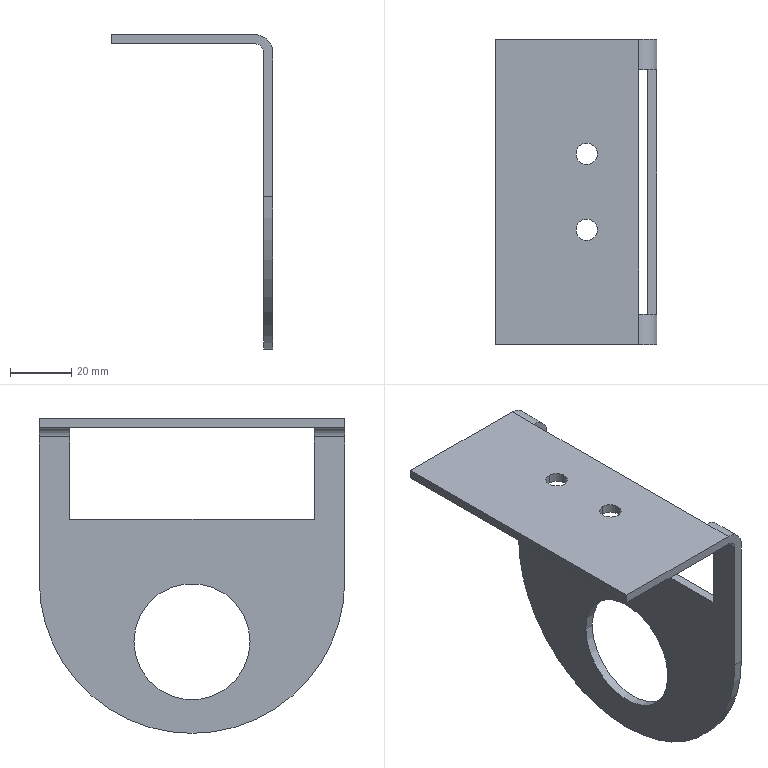Component | SolidWorks | PressureReducingValveHolder-1 | 1 solid | 23 faces | box 53 x 100 x 103 mm | volume 30292 mm3 | cylinder 12 | plane 11 | commonest cylinder face diameters 7 x4 38 x2 6 x2 12 x2 100 x2
STEP:
#1=COLOUR_RGB('',0.7922,0.8196,0.9333);
#2=FILL_AREA_STYLE_COLOUR('',#1);
#3=FILL_AREA_STYLE('',(#2));
#4=SURFACE_STYLE_FILL_AREA(#3);
#5=SURFACE_SIDE_STYLE('',(#4));
#6=SURFACE_STYLE_USAGE(.BOTH.,#5);
#7=PRESENTATION_STYLE_ASSIGNMENT((#6));
#8=CARTESIAN_POINT('',(-6.378,-0.748,-3.366));
#9=VERTEX_POINT('',#8);
#10=CARTESIAN_POINT('',(-6.378,0.748,-3.366));
#11=VERTEX_POINT('',#10);
#12=CARTESIAN_POINT('',(-6.378,0.,-3.366));
#13=DIRECTION('',(-1.,-0.,0.));
#14=DIRECTION('',(0.,1.,0.));
#15=AXIS2_PLACEMENT_3D('',#12,#13,#14);
#16=CIRCLE('',#15,0.748);
#17=EDGE_CURVE('',#9,#11,#16,.T.);
#18=ORIENTED_EDGE('',*,*,#17,.F.);
#19=CARTESIAN_POINT('',(-6.496,-0.748,-3.366));
#20=VERTEX_POINT('',#19);
#21=CARTESIAN_POINT('',(-6.378,-0.748,-3.366));
#22=DIRECTION('',(-1.,-0.,0.));
#23=VECTOR('',#22,39.37);
#24=LINE('',#21,#23);
#25=EDGE_CURVE('',#9,#20,#24,.T.);
#26=ORIENTED_EDGE('',*,*,#25,.T.);
#27=CARTESIAN_POINT('',(-6.496,0.748,-3.366));
#28=VERTEX_POINT('',#27);
#29=CARTESIAN_POINT('',(-6.496,0.,-3.366));
#30=DIRECTION('',(-1.,-0.,0.));
#31=DIRECTION('',(0.,1.,0.));
#32=AXIS2_PLACEMENT_3D('',#29,#30,#31);
#33=CIRCLE('',#32,0.748);
#34=EDGE_CURVE('',#20,#28,#33,.T.);
#35=ORIENTED_EDGE('',*,*,#34,.T.);
#36=CARTESIAN_POINT('',(-6.378,0.748,-3.366));
#37=DIRECTION('',(-1.,-0.,0.));
#38=VECTOR('',#37,39.37);
#39=LINE('',#36,#38);
#40=EDGE_CURVE('',#11,#28,#39,.T.);
#41=ORIENTED_EDGE('',*,*,#40,.F.);
#42=EDGE_LOOP('',(#18,#26,#35,#41));
#43=FACE_OUTER_BOUND('',#42,.T.);
#44=CARTESIAN_POINT('',(-6.378,0.,-3.366));
#45=DIRECTION('',(-1.,-0.,0.));
#46=DIRECTION('',(0.,1.,0.));
#47=AXIS2_PLACEMENT_3D('',#44,#45,#46);
#48=CYLINDRICAL_SURFACE('',#47,0.748);
#49=ADVANCED_FACE('',(#43),#48,.F.);
#50=CARTESIAN_POINT('',(-7.283,-0.628,-0.4921));
#51=VERTEX_POINT('',#50);
#52=CARTESIAN_POINT('',(-7.283,-0.3524,-0.4921));
#53=VERTEX_POINT('',#52);
#54=CARTESIAN_POINT('',(-7.283,-0.4902,-0.4921));
#55=DIRECTION('',(0.,0.,-1.));
#56=DIRECTION('',(0.,1.,0.));
#57=AXIS2_PLACEMENT_3D('',#54,#55,#56);
#58=CIRCLE('',#57,0.1378);
#59=EDGE_CURVE('',#51,#53,#58,.T.);
#60=ORIENTED_EDGE('',*,*,#59,.F.);
#61=CARTESIAN_POINT('',(-7.283,-0.628,-0.6102));
#62=VERTEX_POINT('',#61);
#63=CARTESIAN_POINT('',(-7.283,-0.628,-0.6102));
#64=DIRECTION('',(0.,0.,-1.));
#65=VECTOR('',#64,39.37);
#66=LINE('',#63,#65);
#67=EDGE_CURVE('',#51,#62,#66,.T.);
#68=ORIENTED_EDGE('',*,*,#67,.T.);
#69=CARTESIAN_POINT('',(-7.283,-0.3524,-0.6102));
#70=VERTEX_POINT('',#69);
#71=CARTESIAN_POINT('',(-7.283,-0.4902,-0.6102));
#72=DIRECTION('',(0.,0.,-1.));
#73=DIRECTION('',(0.,1.,0.));
#74=AXIS2_PLACEMENT_3D('',#71,#72,#73);
#75=CIRCLE('',#74,0.1378);
#76=EDGE_CURVE('',#62,#70,#75,.T.);
#77=ORIENTED_EDGE('',*,*,#76,.T.);
#78=CARTESIAN_POINT('',(-7.283,-0.3524,-0.6102));
#79=DIRECTION('',(0.,0.,-1.));
#80=VECTOR('',#79,39.37);
#81=LINE('',#78,#80);
#82=EDGE_CURVE('',#53,#70,#81,.T.);
#83=ORIENTED_EDGE('',*,*,#82,.F.);
#84=EDGE_LOOP('',(#60,#68,#77,#83));
#85=FACE_OUTER_BOUND('',#84,.T.);
#86=CARTESIAN_POINT('',(-7.283,-0.4902,-0.6102));
#87=DIRECTION('',(0.,0.,-1.));
#88=DIRECTION('',(0.,1.,0.));
#89=AXIS2_PLACEMENT_3D('',#86,#87,#88);
#90=CYLINDRICAL_SURFACE('',#89,0.1378);
#91=ADVANCED_FACE('',(#85),#90,.F.);
#92=CARTESIAN_POINT('',(-7.283,0.3524,-0.4921));
#93=VERTEX_POINT('',#92);
#94=CARTESIAN_POINT('',(-7.283,0.628,-0.4921));
#95=VERTEX_POINT('',#94);
#96=CARTESIAN_POINT('',(-7.283,0.4902,-0.4921));
#97=DIRECTION('',(0.,0.,-1.));
#98=DIRECTION('',(0.,1.,0.));
#99=AXIS2_PLACEMENT_3D('',#96,#97,#98);
#100=CIRCLE('',#99,0.1378);
#101=EDGE_CURVE('',#93,#95,#100,.T.);
#102=ORIENTED_EDGE('',*,*,#101,.F.);
#103=CARTESIAN_POINT('',(-7.283,0.3524,-0.6102));
#104=VERTEX_POINT('',#103);
#105=CARTESIAN_POINT('',(-7.283,0.3524,-0.6102));
#106=DIRECTION('',(0.,0.,-1.));
#107=VECTOR('',#106,39.37);
#108=LINE('',#105,#107);
#109=EDGE_CURVE('',#93,#104,#108,.T.);
#110=ORIENTED_EDGE('',*,*,#109,.T.);
#111=CARTESIAN_POINT('',(-7.283,0.628,-0.6102));
#112=VERTEX_POINT('',#111);
#113=CARTESIAN_POINT('',(-7.283,0.4902,-0.6102));
#114=DIRECTION('',(0.,0.,-1.));
#115=DIRECTION('',(0.,1.,0.));
#116=AXIS2_PLACEMENT_3D('',#113,#114,#115);
#117=CIRCLE('',#116,0.1378);
#118=EDGE_CURVE('',#104,#112,#117,.T.);
#119=ORIENTED_EDGE('',*,*,#118,.T.);
#120=CARTESIAN_POINT('',(-7.283,0.628,-0.6102));
#121=DIRECTION('',(0.,0.,-1.));
#122=VECTOR('',#121,39.37);
#123=LINE('',#120,#122);
#124=EDGE_CURVE('',#95,#112,#123,.T.);
#125=ORIENTED_EDGE('',*,*,#124,.F.);
#126=EDGE_LOOP('',(#102,#110,#119,#125));
#127=FACE_OUTER_BOUND('',#126,.T.);
#128=CARTESIAN_POINT('',(-7.283,0.4902,-0.6102));
#129=DIRECTION('',(0.,0.,-1.));
#130=DIRECTION('',(0.,1.,0.));
#131=AXIS2_PLACEMENT_3D('',#128,#129,#130);
#132=CYLINDRICAL_SURFACE('',#131,0.1378);
#133=ADVANCED_FACE('',(#127),#132,.F.);
#134=CARTESIAN_POINT('',(-6.496,-1.575,-0.7283));
#135=VERTEX_POINT('',#134);
#136=CARTESIAN_POINT('',(-6.614,-1.575,-0.6102));
#137=VERTEX_POINT('',#136);
#138=CARTESIAN_POINT('',(-6.614,-1.575,-0.7283));
#139=DIRECTION('',(0.,-1.,0.));
#140=DIRECTION('',(0.,0.,-1.));
#141=AXIS2_PLACEMENT_3D('',#138,#139,#140);
#142=CIRCLE('',#141,0.1181);
#143=EDGE_CURVE('',#135,#137,#142,.T.);
#144=ORIENTED_EDGE('',*,*,#143,.F.);
#145=CARTESIAN_POINT('',(-6.496,-1.969,-0.7283));
#146=VERTEX_POINT('',#145);
#147=CARTESIAN_POINT('',(-6.496,-1.969,-0.7283));
#148=DIRECTION('',(-0.,1.,0.));
#149=VECTOR('',#148,39.37);
#150=LINE('',#147,#149);
#151=EDGE_CURVE('',#146,#135,#150,.T.);
#152=ORIENTED_EDGE('',*,*,#151,.F.);
#153=CARTESIAN_POINT('',(-6.614,-1.969,-0.6102));
#154=VERTEX_POINT('',#153);
#155=CARTESIAN_POINT('',(-6.614,-1.969,-0.7283));
#156=DIRECTION('',(0.,-1.,0.));
#157=DIRECTION('',(0.,0.,-1.));
#158=AXIS2_PLACEMENT_3D('',#155,#156,#157);
#159=CIRCLE('',#158,0.1181);
#160=EDGE_CURVE('',#146,#154,#159,.T.);
#161=ORIENTED_EDGE('',*,*,#160,.T.);
#162=CARTESIAN_POINT('',(-6.614,-1.969,-0.6102));
#163=DIRECTION('',(-0.,1.,0.));
#164=VECTOR('',#163,39.37);
#165=LINE('',#162,#164);
#166=EDGE_CURVE('',#154,#137,#165,.T.);
#167=ORIENTED_EDGE('',*,*,#166,.T.);
#168=EDGE_LOOP('',(#144,#152,#161,#167));
#169=FACE_OUTER_BOUND('',#168,.T.);
#170=CARTESIAN_POINT('',(-6.614,-1.969,-0.7283));
#171=DIRECTION('',(-0.,1.,0.));
#172=DIRECTION('',(0.,0.,1.));
#173=AXIS2_PLACEMENT_3D('',#170,#171,#172);
#174=CYLINDRICAL_SURFACE('',#173,0.1181);
#175=ADVANCED_FACE('',(#169),#174,.F.);
#176=CARTESIAN_POINT('',(-6.378,-1.969,-0.7283));
#177=VERTEX_POINT('',#176);
#178=CARTESIAN_POINT('',(-6.378,-1.575,-0.7283));
#179=VERTEX_POINT('',#178);
#180=CARTESIAN_POINT('',(-6.378,-1.969,-0.7283));
#181=DIRECTION('',(-0.,1.,0.));
#182=VECTOR('',#181,39.37);
#183=LINE('',#180,#182);
#184=EDGE_CURVE('',#177,#179,#183,.T.);
#185=ORIENTED_EDGE('',*,*,#184,.T.);
#186=CARTESIAN_POINT('',(-6.614,-1.575,-0.4921));
#187=VERTEX_POINT('',#186);
#188=CARTESIAN_POINT('',(-6.614,-1.575,-0.7283));
#189=DIRECTION('',(0.,-1.,0.));
#190=DIRECTION('',(0.,0.,-1.));
#191=AXIS2_PLACEMENT_3D('',#188,#189,#190);
#192=CIRCLE('',#191,0.2362);
#193=EDGE_CURVE('',#179,#187,#192,.T.);
#194=ORIENTED_EDGE('',*,*,#193,.T.);
#195=CARTESIAN_POINT('',(-6.614,-1.969,-0.4921));
#196=VERTEX_POINT('',#195);
#197=CARTESIAN_POINT('',(-6.614,-1.969,-0.4921));
#198=DIRECTION('',(-0.,1.,0.));
#199=VECTOR('',#198,39.37);
#200=LINE('',#197,#199);
#201=EDGE_CURVE('',#196,#187,#200,.T.);
#202=ORIENTED_EDGE('',*,*,#201,.F.);
#203=CARTESIAN_POINT('',(-6.614,-1.969,-0.7283));
#204=DIRECTION('',(0.,-1.,0.));
#205=DIRECTION('',(0.,0.,-1.));
#206=AXIS2_PLACEMENT_3D('',#203,#204,#205);
#207=CIRCLE('',#206,0.2362);
#208=EDGE_CURVE('',#177,#196,#207,.T.);
#209=ORIENTED_EDGE('',*,*,#208,.F.);
#210=EDGE_LOOP('',(#185,#194,#202,#209));
#211=FACE_OUTER_BOUND('',#210,.T.);
#212=CARTESIAN_POINT('',(-6.614,-1.969,-0.7283));
#213=DIRECTION('',(-0.,1.,0.));
#214=DIRECTION('',(0.,0.,1.));
#215=AXIS2_PLACEMENT_3D('',#212,#213,#214);
#216=CYLINDRICAL_SURFACE('',#215,0.2362);
#217=ADVANCED_FACE('',(#211),#216,.T.);
#218=CARTESIAN_POINT('',(-7.283,-0.4902,-0.4921));
#219=DIRECTION('',(0.,0.,-1.));
#220=DIRECTION('',(0.,1.,0.));
#221=AXIS2_PLACEMENT_3D('',#218,#219,#220);
#222=CIRCLE('',#221,0.1378);
#223=EDGE_CURVE('',#53,#51,#222,.T.);
#224=ORIENTED_EDGE('',*,*,#223,.T.);
#225=ORIENTED_EDGE('',*,*,#59,.T.);
#226=EDGE_LOOP('',(#224,#225));
#227=FACE_BOUND('',#226,.T.);
#228=CARTESIAN_POINT('',(-7.283,0.4902,-0.4921));
#229=DIRECTION('',(0.,0.,-1.));
#230=DIRECTION('',(0.,1.,0.));
#231=AXIS2_PLACEMENT_3D('',#228,#229,#230);
#232=CIRCLE('',#231,0.1378);
#233=EDGE_CURVE('',#95,#93,#232,.T.);
#234=ORIENTED_EDGE('',*,*,#233,.T.);
#235=ORIENTED_EDGE('',*,*,#101,.T.);
#236=EDGE_LOOP('',(#234,#235));
#237=FACE_BOUND('',#236,.T.);
#238=CARTESIAN_POINT('',(-6.614,1.969,-0.4921));
#239=VERTEX_POINT('',#238);
#240=CARTESIAN_POINT('',(-8.465,1.969,-0.4921));
#241=VERTEX_POINT('',#240);
#242=CARTESIAN_POINT('',(-6.614,1.969,-0.4921));
#243=DIRECTION('',(-1.,-0.,0.));
#244=VECTOR('',#243,39.37);
#245=LINE('',#242,#244);
#246=EDGE_CURVE('',#239,#241,#245,.T.);
#247=ORIENTED_EDGE('',*,*,#246,.T.);
#248=CARTESIAN_POINT('',(-8.465,-1.969,-0.4921));
#249=VERTEX_POINT('',#248);
#250=CARTESIAN_POINT('',(-8.465,-1.969,-0.4921));
#251=DIRECTION('',(-0.,1.,0.));
#252=VECTOR('',#251,39.37);
#253=LINE('',#250,#252);
#254=EDGE_CURVE('',#249,#241,#253,.T.);
#255=ORIENTED_EDGE('',*,*,#254,.F.);
#256=CARTESIAN_POINT('',(-6.614,-1.969,-0.4921));
#257=DIRECTION('',(-1.,-0.,0.));
#258=VECTOR('',#257,39.37);
#259=LINE('',#256,#258);
#260=EDGE_CURVE('',#196,#249,#259,.T.);
#261=ORIENTED_EDGE('',*,*,#260,.F.);
#262=ORIENTED_EDGE('',*,*,#201,.T.);
#263=CARTESIAN_POINT('',(-6.614,1.575,-0.4921));
#264=VERTEX_POINT('',#263);
#265=CARTESIAN_POINT('',(-6.614,-1.969,-0.4921));
#266=DIRECTION('',(-0.,1.,0.));
#267=VECTOR('',#266,39.37);
#268=LINE('',#265,#267);
#269=EDGE_CURVE('',#187,#264,#268,.T.);
#270=ORIENTED_EDGE('',*,*,#269,.T.);
#271=CARTESIAN_POINT('',(-6.614,-1.969,-0.4921));
#272=DIRECTION('',(-0.,1.,0.));
#273=VECTOR('',#272,39.37);
#274=LINE('',#271,#273);
#275=EDGE_CURVE('',#264,#239,#274,.T.);
#276=ORIENTED_EDGE('',*,*,#275,.T.);
#277=EDGE_LOOP('',(#247,#255,#261,#262,#270,#276));
#278=FACE_OUTER_BOUND('',#277,.T.);
#279=CARTESIAN_POINT('',(-6.614,-1.969,-0.4921));
#280=DIRECTION('',(0.,0.,-1.));
#281=DIRECTION('',(-0.,1.,0.));
#282=AXIS2_PLACEMENT_3D('',#279,#280,#281);
#283=PLANE('',#282);
#284=ADVANCED_FACE('',(#227,#237,#278),#283,.F.);
#285=CARTESIAN_POINT('',(-8.465,1.969,-0.6102));
#286=VERTEX_POINT('',#285);
#287=CARTESIAN_POINT('',(-8.465,1.969,-0.6102));
#288=DIRECTION('',(0.,0.,1.));
#289=VECTOR('',#288,39.37);
#290=LINE('',#287,#289);
#291=EDGE_CURVE('',#286,#241,#290,.T.);
#292=ORIENTED_EDGE('',*,*,#291,.F.);
#293=CARTESIAN_POINT('',(-8.465,-1.969,-0.6102));
#294=VERTEX_POINT('',#293);
#295=CARTESIAN_POINT('',(-8.465,-1.969,-0.6102));
#296=DIRECTION('',(-0.,1.,0.));
#297=VECTOR('',#296,39.37);
#298=LINE('',#295,#297);
#299=EDGE_CURVE('',#294,#286,#298,.T.);
#300=ORIENTED_EDGE('',*,*,#299,.F.);
#301=CARTESIAN_POINT('',(-8.465,-1.969,-0.6102));
#302=DIRECTION('',(0.,0.,1.));
#303=VECTOR('',#302,39.37);
#304=LINE('',#301,#303);
#305=EDGE_CURVE('',#294,#249,#304,.T.);
#306=ORIENTED_EDGE('',*,*,#305,.T.);
#307=ORIENTED_EDGE('',*,*,#254,.T.);
#308=EDGE_LOOP('',(#292,#300,#306,#307));
#309=FACE_OUTER_BOUND('',#308,.T.);
#310=CARTESIAN_POINT('',(-8.465,-1.969,-0.6102));
#311=DIRECTION('',(-1.,-0.,0.));
#312=DIRECTION('',(-0.,1.,0.));
#313=AXIS2_PLACEMENT_3D('',#310,#311,#312);
#314=PLANE('',#313);
#315=ADVANCED_FACE('',(#309),#314,.T.);
#316=CARTESIAN_POINT('',(-7.283,-0.4902,-0.6102));
#317=DIRECTION('',(0.,0.,-1.));
#318=DIRECTION('',(0.,1.,0.));
#319=AXIS2_PLACEMENT_3D('',#316,#317,#318);
#320=CIRCLE('',#319,0.1378);
#321=EDGE_CURVE('',#70,#62,#320,.T.);
#322=ORIENTED_EDGE('',*,*,#321,.F.);
#323=ORIENTED_EDGE('',*,*,#76,.F.);
#324=EDGE_LOOP('',(#322,#323));
#325=FACE_BOUND('',#324,.T.);
#326=CARTESIAN_POINT('',(-7.283,0.4902,-0.6102));
#327=DIRECTION('',(0.,0.,-1.));
#328=DIRECTION('',(0.,1.,0.));
#329=AXIS2_PLACEMENT_3D('',#326,#327,#328);
#330=CIRCLE('',#329,0.1378);
#331=EDGE_CURVE('',#112,#104,#330,.T.);
#332=ORIENTED_EDGE('',*,*,#331,.F.);
#333=ORIENTED_EDGE('',*,*,#118,.F.);
#334=EDGE_LOOP('',(#332,#333));
#335=FACE_BOUND('',#334,.T.);
#336=CARTESIAN_POINT('',(-6.614,1.969,-0.6102));
#337=VERTEX_POINT('',#336);
#338=CARTESIAN_POINT('',(-6.614,1.969,-0.6102));
#339=DIRECTION('',(-1.,-0.,0.));
#340=VECTOR('',#339,39.37);
#341=LINE('',#338,#340);
#342=EDGE_CURVE('',#337,#286,#341,.T.);
#343=ORIENTED_EDGE('',*,*,#342,.F.);
#344=CARTESIAN_POINT('',(-6.614,1.575,-0.6102));
#345=VERTEX_POINT('',#344);
#346=CARTESIAN_POINT('',(-6.614,-1.969,-0.6102));
#347=DIRECTION('',(-0.,1.,0.));
#348=VECTOR('',#347,39.37);
#349=LINE('',#346,#348);
#350=EDGE_CURVE('',#345,#337,#349,.T.);
#351=ORIENTED_EDGE('',*,*,#350,.F.);
#352=CARTESIAN_POINT('',(-6.614,-1.969,-0.6102));
#353=DIRECTION('',(0.,-1.,0.));
#354=VECTOR('',#353,39.37);
#355=LINE('',#352,#354);
#356=EDGE_CURVE('',#345,#137,#355,.T.);
#357=ORIENTED_EDGE('',*,*,#356,.T.);
#358=ORIENTED_EDGE('',*,*,#166,.F.);
#359=CARTESIAN_POINT('',(-6.614,-1.969,-0.6102));
#360=DIRECTION('',(-1.,-0.,0.));
#361=VECTOR('',#360,39.37);
#362=LINE('',#359,#361);
#363=EDGE_CURVE('',#154,#294,#362,.T.);
#364=ORIENTED_EDGE('',*,*,#363,.T.);
#365=ORIENTED_EDGE('',*,*,#299,.T.);
#366=EDGE_LOOP('',(#343,#351,#357,#358,#364,#365));
#367=FACE_OUTER_BOUND('',#366,.T.);
#368=CARTESIAN_POINT('',(-6.614,-1.969,-0.6102));
#369=DIRECTION('',(0.,0.,-1.));
#370=DIRECTION('',(-0.,1.,0.));
#371=AXIS2_PLACEMENT_3D('',#368,#369,#370);
#372=PLANE('',#371);
#373=ADVANCED_FACE('',(#325,#335,#367),#372,.T.);
#374=CARTESIAN_POINT('',(-6.496,1.575,-0.7283));
#375=VERTEX_POINT('',#374);
#376=CARTESIAN_POINT('',(-6.614,1.575,-0.7283));
#377=DIRECTION('',(-0.,1.,0.));
#378=DIRECTION('',(0.,0.,1.));
#379=AXIS2_PLACEMENT_3D('',#376,#377,#378);
#380=CIRCLE('',#379,0.1181);
#381=EDGE_CURVE('',#345,#375,#380,.T.);
#382=ORIENTED_EDGE('',*,*,#381,.F.);
#383=ORIENTED_EDGE('',*,*,#350,.T.);
#384=CARTESIAN_POINT('',(-6.496,1.969,-0.7283));
#385=VERTEX_POINT('',#384);
#386=CARTESIAN_POINT('',(-6.614,1.969,-0.7283));
#387=DIRECTION('',(0.,-1.,0.));
#388=DIRECTION('',(0.,0.,-1.));
#389=AXIS2_PLACEMENT_3D('',#386,#387,#388);
#390=CIRCLE('',#389,0.1181);
#391=EDGE_CURVE('',#385,#337,#390,.T.);
#392=ORIENTED_EDGE('',*,*,#391,.F.);
#393=CARTESIAN_POINT('',(-6.496,-1.969,-0.7283));
#394=DIRECTION('',(-0.,1.,0.));
#395=VECTOR('',#394,39.37);
#396=LINE('',#393,#395);
#397=EDGE_CURVE('',#375,#385,#396,.T.);
#398=ORIENTED_EDGE('',*,*,#397,.F.);
#399=EDGE_LOOP('',(#382,#383,#392,#398));
#400=FACE_OUTER_BOUND('',#399,.T.);
#401=CARTESIAN_POINT('',(-6.614,-1.969,-0.7283));
#402=DIRECTION('',(-0.,1.,0.));
#403=DIRECTION('',(0.,0.,1.));
#404=AXIS2_PLACEMENT_3D('',#401,#402,#403);
#405=CYLINDRICAL_SURFACE('',#404,0.1181);
#406=ADVANCED_FACE('',(#400),#405,.F.);
#407=CARTESIAN_POINT('',(-6.496,0.,-3.366));
#408=DIRECTION('',(-1.,-0.,0.));
#409=DIRECTION('',(0.,1.,0.));
#410=AXIS2_PLACEMENT_3D('',#407,#408,#409);
#411=CIRCLE('',#410,0.748);
#412=EDGE_CURVE('',#28,#20,#411,.T.);
#413=ORIENTED_EDGE('',*,*,#412,.F.);
#414=ORIENTED_EDGE('',*,*,#34,.F.);
#415=EDGE_LOOP('',(#413,#414));
#416=FACE_BOUND('',#415,.T.);
#417=CARTESIAN_POINT('',(-6.496,1.969,-2.579));
#418=VERTEX_POINT('',#417);
#419=CARTESIAN_POINT('',(-6.496,1.969,-0.7283));
#420=DIRECTION('',(0.,0.,1.));
#421=VECTOR('',#420,39.37);
#422=LINE('',#419,#421);
#423=EDGE_CURVE('',#418,#385,#422,.T.);
#424=ORIENTED_EDGE('',*,*,#423,.F.);
#425=CARTESIAN_POINT('',(-6.496,0.,-4.547));
#426=VERTEX_POINT('',#425);
#427=CARTESIAN_POINT('',(-6.496,0.,-2.579));
#428=DIRECTION('',(-1.,-0.,0.));
#429=DIRECTION('',(0.,1.,0.));
#430=AXIS2_PLACEMENT_3D('',#427,#428,#429);
#431=CIRCLE('',#430,1.969);
#432=EDGE_CURVE('',#418,#426,#431,.T.);
#433=ORIENTED_EDGE('',*,*,#432,.T.);
#434=CARTESIAN_POINT('',(-6.496,-1.969,-2.579));
#435=VERTEX_POINT('',#434);
#436=CARTESIAN_POINT('',(-6.496,0.,-2.579));
#437=DIRECTION('',(-1.,-0.,0.));
#438=DIRECTION('',(0.,1.,0.));
#439=AXIS2_PLACEMENT_3D('',#436,#437,#438);
#440=CIRCLE('',#439,1.969);
#441=EDGE_CURVE('',#426,#435,#440,.T.);
#442=ORIENTED_EDGE('',*,*,#441,.T.);
#443=CARTESIAN_POINT('',(-6.496,-1.969,-0.7283));
#444=DIRECTION('',(0.,0.,1.));
#445=VECTOR('',#444,39.37);
#446=LINE('',#443,#445);
#447=EDGE_CURVE('',#435,#146,#446,.T.);
#448=ORIENTED_EDGE('',*,*,#447,.T.);
#449=ORIENTED_EDGE('',*,*,#151,.T.);
#450=CARTESIAN_POINT('',(-6.496,-1.575,-1.791));
#451=VERTEX_POINT('',#450);
#452=CARTESIAN_POINT('',(-6.496,-1.575,-0.7283));
#453=DIRECTION('',(0.,0.,1.));
#454=VECTOR('',#453,39.37);
#455=LINE('',#452,#454);
#456=EDGE_CURVE('',#451,#135,#455,.T.);
#457=ORIENTED_EDGE('',*,*,#456,.F.);
#458=CARTESIAN_POINT('',(-6.496,1.575,-1.791));
#459=VERTEX_POINT('',#458);
#460=CARTESIAN_POINT('',(-6.496,-1.969,-1.791));
#461=DIRECTION('',(0.,-1.,-0.));
#462=VECTOR('',#461,39.37);
#463=LINE('',#460,#462);
#464=EDGE_CURVE('',#459,#451,#463,.T.);
#465=ORIENTED_EDGE('',*,*,#464,.F.);
#466=CARTESIAN_POINT('',(-6.496,1.575,-0.7283));
#467=DIRECTION('',(0.,0.,-1.));
#468=VECTOR('',#467,39.37);
#469=LINE('',#466,#468);
#470=EDGE_CURVE('',#375,#459,#469,.T.);
#471=ORIENTED_EDGE('',*,*,#470,.F.);
#472=ORIENTED_EDGE('',*,*,#397,.T.);
#473=EDGE_LOOP('',(#424,#433,#442,#448,#449,#457,#465,#471,#472));
#474=FACE_OUTER_BOUND('',#473,.T.);
#475=CARTESIAN_POINT('',(-6.496,-1.969,-0.7283));
#476=DIRECTION('',(-1.,-0.,0.));
#477=DIRECTION('',(-0.,1.,0.));
#478=AXIS2_PLACEMENT_3D('',#475,#476,#477);
#479=PLANE('',#478);
#480=ADVANCED_FACE('',(#416,#474),#479,.T.);
#481=CARTESIAN_POINT('',(-6.378,0.,-3.366));
#482=DIRECTION('',(-1.,-0.,0.));
#483=DIRECTION('',(0.,1.,0.));
#484=AXIS2_PLACEMENT_3D('',#481,#482,#483);
#485=CIRCLE('',#484,0.748);
#486=EDGE_CURVE('',#11,#9,#485,.T.);
#487=ORIENTED_EDGE('',*,*,#486,.T.);
#488=ORIENTED_EDGE('',*,*,#17,.T.);
#489=EDGE_LOOP('',(#487,#488));
#490=FACE_BOUND('',#489,.T.);
#491=CARTESIAN_POINT('',(-6.378,-1.969,-2.579));
#492=VERTEX_POINT('',#491);
#493=CARTESIAN_POINT('',(-6.378,0.,-4.547));
#494=VERTEX_POINT('',#493);
#495=CARTESIAN_POINT('',(-6.378,0.,-2.579));
#496=DIRECTION('',(1.,0.,0.));
#497=DIRECTION('',(0.,1.,0.));
#498=AXIS2_PLACEMENT_3D('',#495,#496,#497);
#499=CIRCLE('',#498,1.969);
#500=EDGE_CURVE('',#492,#494,#499,.T.);
#501=ORIENTED_EDGE('',*,*,#500,.T.);
#502=CARTESIAN_POINT('',(-6.378,1.969,-2.579));
#503=VERTEX_POINT('',#502);
#504=CARTESIAN_POINT('',(-6.378,0.,-2.579));
#505=DIRECTION('',(1.,0.,0.));
#506=DIRECTION('',(0.,1.,0.));
#507=AXIS2_PLACEMENT_3D('',#504,#505,#506);
#508=CIRCLE('',#507,1.969);
#509=EDGE_CURVE('',#494,#503,#508,.T.);
#510=ORIENTED_EDGE('',*,*,#509,.T.);
#511=CARTESIAN_POINT('',(-6.378,1.969,-0.7283));
#512=VERTEX_POINT('',#511);
#513=CARTESIAN_POINT('',(-6.378,1.969,-0.7283));
#514=DIRECTION('',(0.,0.,1.));
#515=VECTOR('',#514,39.37);
#516=LINE('',#513,#515);
#517=EDGE_CURVE('',#503,#512,#516,.T.);
#518=ORIENTED_EDGE('',*,*,#517,.T.);
#519=CARTESIAN_POINT('',(-6.378,1.575,-0.7283));
#520=VERTEX_POINT('',#519);
#521=CARTESIAN_POINT('',(-6.378,-1.969,-0.7283));
#522=DIRECTION('',(-0.,1.,0.));
#523=VECTOR('',#522,39.37);
#524=LINE('',#521,#523);
#525=EDGE_CURVE('',#520,#512,#524,.T.);
#526=ORIENTED_EDGE('',*,*,#525,.F.);
#527=CARTESIAN_POINT('',(-6.378,1.575,-1.791));
#528=VERTEX_POINT('',#527);
#529=CARTESIAN_POINT('',(-6.378,1.575,0.5709));
#530=DIRECTION('',(0.,0.,1.));
#531=VECTOR('',#530,39.37);
#532=LINE('',#529,#531);
#533=EDGE_CURVE('',#528,#520,#532,.T.);
#534=ORIENTED_EDGE('',*,*,#533,.F.);
#535=CARTESIAN_POINT('',(-6.378,-1.575,-1.791));
#536=VERTEX_POINT('',#535);
#537=CARTESIAN_POINT('',(-6.378,1.575,-1.791));
#538=DIRECTION('',(-0.,1.,0.));
#539=VECTOR('',#538,39.37);
#540=LINE('',#537,#539);
#541=EDGE_CURVE('',#536,#528,#540,.T.);
#542=ORIENTED_EDGE('',*,*,#541,.F.);
#543=CARTESIAN_POINT('',(-6.378,-1.575,0.5709));
#544=DIRECTION('',(0.,0.,-1.));
#545=VECTOR('',#544,39.37);
#546=LINE('',#543,#545);
#547=EDGE_CURVE('',#179,#536,#546,.T.);
#548=ORIENTED_EDGE('',*,*,#547,.F.);
#549=ORIENTED_EDGE('',*,*,#184,.F.);
#550=CARTESIAN_POINT('',(-6.378,-1.969,-0.7283));
#551=DIRECTION('',(0.,0.,1.));
#552=VECTOR('',#551,39.37);
#553=LINE('',#550,#552);
#554=EDGE_CURVE('',#492,#177,#553,.T.);
#555=ORIENTED_EDGE('',*,*,#554,.F.);
#556=EDGE_LOOP('',(#501,#510,#518,#526,#534,#542,#548,#549,#555));
#557=FACE_OUTER_BOUND('',#556,.T.);
#558=CARTESIAN_POINT('',(-6.378,-1.969,-0.7283));
#559=DIRECTION('',(-1.,-0.,0.));
#560=DIRECTION('',(-0.,1.,0.));
#561=AXIS2_PLACEMENT_3D('',#558,#559,#560);
#562=PLANE('',#561);
#563=ADVANCED_FACE('',(#490,#557),#562,.F.);
#564=ORIENTED_EDGE('',*,*,#275,.F.);
#565=CARTESIAN_POINT('',(-6.614,1.575,-0.7283));
#566=DIRECTION('',(-0.,1.,0.));
#567=DIRECTION('',(0.,0.,1.));
#568=AXIS2_PLACEMENT_3D('',#565,#566,#567);
#569=CIRCLE('',#568,0.2362);
#570=EDGE_CURVE('',#264,#520,#569,.T.);
#571=ORIENTED_EDGE('',*,*,#570,.T.);
#572=ORIENTED_EDGE('',*,*,#525,.T.);
#573=CARTESIAN_POINT('',(-6.614,1.969,-0.7283));
#574=DIRECTION('',(0.,-1.,0.));
#575=DIRECTION('',(0.,0.,-1.));
#576=AXIS2_PLACEMENT_3D('',#573,#574,#575);
#577=CIRCLE('',#576,0.2362);
#578=EDGE_CURVE('',#512,#239,#577,.T.);
#579=ORIENTED_EDGE('',*,*,#578,.T.);
#580=EDGE_LOOP('',(#564,#571,#572,#579));
#581=FACE_OUTER_BOUND('',#580,.T.);
#582=CARTESIAN_POINT('',(-6.614,-1.969,-0.7283));
#583=DIRECTION('',(-0.,1.,0.));
#584=DIRECTION('',(0.,0.,1.));
#585=AXIS2_PLACEMENT_3D('',#582,#583,#584);
#586=CYLINDRICAL_SURFACE('',#585,0.2362);
#587=ADVANCED_FACE('',(#581),#586,.T.);
#588=ORIENTED_EDGE('',*,*,#447,.F.);
#589=CARTESIAN_POINT('',(-6.614,-1.969,-2.579));
#590=DIRECTION('',(1.,0.,0.));
#591=VECTOR('',#590,39.37);
#592=LINE('',#589,#591);
#593=EDGE_CURVE('',#435,#492,#592,.T.);
#594=ORIENTED_EDGE('',*,*,#593,.T.);
#595=ORIENTED_EDGE('',*,*,#554,.T.);
#596=ORIENTED_EDGE('',*,*,#208,.T.);
#597=ORIENTED_EDGE('',*,*,#260,.T.);
#598=ORIENTED_EDGE('',*,*,#305,.F.);
#599=ORIENTED_EDGE('',*,*,#363,.F.);
#600=ORIENTED_EDGE('',*,*,#160,.F.);
#601=EDGE_LOOP('',(#588,#594,#595,#596,#597,#598,#599,#600));
#602=FACE_OUTER_BOUND('',#601,.T.);
#603=CARTESIAN_POINT('',(-6.614,-1.969,-0.7283));
#604=DIRECTION('',(0.,-1.,0.));
#605=DIRECTION('',(0.,0.,-1.));
#606=AXIS2_PLACEMENT_3D('',#603,#604,#605);
#607=PLANE('',#606);
#608=ADVANCED_FACE('',(#602),#607,.T.);
#609=ORIENTED_EDGE('',*,*,#517,.F.);
#610=CARTESIAN_POINT('',(-6.496,1.969,-2.579));
#611=DIRECTION('',(-1.,-0.,0.));
#612=VECTOR('',#611,39.37);
#613=LINE('',#610,#612);
#614=EDGE_CURVE('',#503,#418,#613,.T.);
#615=ORIENTED_EDGE('',*,*,#614,.T.);
#616=ORIENTED_EDGE('',*,*,#423,.T.);
#617=ORIENTED_EDGE('',*,*,#391,.T.);
#618=ORIENTED_EDGE('',*,*,#342,.T.);
#619=ORIENTED_EDGE('',*,*,#291,.T.);
#620=ORIENTED_EDGE('',*,*,#246,.F.);
#621=ORIENTED_EDGE('',*,*,#578,.F.);
#622=EDGE_LOOP('',(#609,#615,#616,#617,#618,#619,#620,#621));
#623=FACE_OUTER_BOUND('',#622,.T.);
#624=CARTESIAN_POINT('',(-6.614,1.969,-0.7283));
#625=DIRECTION('',(0.,-1.,0.));
#626=DIRECTION('',(0.,0.,-1.));
#627=AXIS2_PLACEMENT_3D('',#624,#625,#626);
#628=PLANE('',#627);
#629=ADVANCED_FACE('',(#623),#628,.F.);
#630=ORIENTED_EDGE('',*,*,#109,.F.);
#631=ORIENTED_EDGE('',*,*,#233,.F.);
#632=ORIENTED_EDGE('',*,*,#124,.T.);
#633=ORIENTED_EDGE('',*,*,#331,.T.);
#634=EDGE_LOOP('',(#630,#631,#632,#633));
#635=FACE_OUTER_BOUND('',#634,.T.);
#636=CARTESIAN_POINT('',(-7.283,0.4902,-0.6102));
#637=DIRECTION('',(0.,0.,-1.));
#638=DIRECTION('',(0.,1.,0.));
#639=AXIS2_PLACEMENT_3D('',#636,#637,#638);
#640=CYLINDRICAL_SURFACE('',#639,0.1378);
#641=ADVANCED_FACE('',(#635),#640,.F.);
#642=ORIENTED_EDGE('',*,*,#67,.F.);
#643=ORIENTED_EDGE('',*,*,#223,.F.);
#644=ORIENTED_EDGE('',*,*,#82,.T.);
#645=ORIENTED_EDGE('',*,*,#321,.T.);
#646=EDGE_LOOP('',(#642,#643,#644,#645));
#647=FACE_OUTER_BOUND('',#646,.T.);
#648=CARTESIAN_POINT('',(-7.283,-0.4902,-0.6102));
#649=DIRECTION('',(0.,0.,-1.));
#650=DIRECTION('',(0.,1.,0.));
#651=AXIS2_PLACEMENT_3D('',#648,#649,#650);
#652=CYLINDRICAL_SURFACE('',#651,0.1378);
#653=ADVANCED_FACE('',(#647),#652,.F.);
#654=ORIENTED_EDGE('',*,*,#143,.T.);
#655=CARTESIAN_POINT('',(-6.614,-1.575,0.5709));
#656=DIRECTION('',(0.,0.,-1.));
#657=VECTOR('',#656,39.37);
#658=LINE('',#655,#657);
#659=EDGE_CURVE('',#187,#137,#658,.T.);
#660=ORIENTED_EDGE('',*,*,#659,.F.);
#661=ORIENTED_EDGE('',*,*,#193,.F.);
#662=ORIENTED_EDGE('',*,*,#547,.T.);
#663=CARTESIAN_POINT('',(-6.614,-1.575,-1.791));
#664=DIRECTION('',(1.,0.,0.));
#665=VECTOR('',#664,39.37);
#666=LINE('',#663,#665);
#667=EDGE_CURVE('',#451,#536,#666,.T.);
#668=ORIENTED_EDGE('',*,*,#667,.F.);
#669=ORIENTED_EDGE('',*,*,#456,.T.);
#670=EDGE_LOOP('',(#654,#660,#661,#662,#668,#669));
#671=FACE_OUTER_BOUND('',#670,.T.);
#672=CARTESIAN_POINT('',(-6.614,-1.575,0.5709));
#673=DIRECTION('',(0.,-1.,0.));
#674=DIRECTION('',(0.,0.,-1.));
#675=AXIS2_PLACEMENT_3D('',#672,#673,#674);
#676=PLANE('',#675);
#677=ADVANCED_FACE('',(#671),#676,.F.);
#678=ORIENTED_EDGE('',*,*,#381,.T.);
#679=ORIENTED_EDGE('',*,*,#470,.T.);
#680=CARTESIAN_POINT('',(-6.614,1.575,-1.791));
#681=DIRECTION('',(1.,0.,0.));
#682=VECTOR('',#681,39.37);
#683=LINE('',#680,#682);
#684=EDGE_CURVE('',#459,#528,#683,.T.);
#685=ORIENTED_EDGE('',*,*,#684,.T.);
#686=ORIENTED_EDGE('',*,*,#533,.T.);
#687=ORIENTED_EDGE('',*,*,#570,.F.);
#688=CARTESIAN_POINT('',(-6.614,1.575,0.5709));
#689=DIRECTION('',(0.,0.,1.));
#690=VECTOR('',#689,39.37);
#691=LINE('',#688,#690);
#692=EDGE_CURVE('',#345,#264,#691,.T.);
#693=ORIENTED_EDGE('',*,*,#692,.F.);
#694=EDGE_LOOP('',(#678,#679,#685,#686,#687,#693));
#695=FACE_OUTER_BOUND('',#694,.T.);
#696=CARTESIAN_POINT('',(-6.614,1.575,0.5709));
#697=DIRECTION('',(-0.,1.,0.));
#698=DIRECTION('',(0.,0.,1.));
#699=AXIS2_PLACEMENT_3D('',#696,#697,#698);
#700=PLANE('',#699);
#701=ADVANCED_FACE('',(#695),#700,.F.);
#702=ORIENTED_EDGE('',*,*,#692,.T.);
#703=ORIENTED_EDGE('',*,*,#269,.F.);
#704=ORIENTED_EDGE('',*,*,#659,.T.);
#705=ORIENTED_EDGE('',*,*,#356,.F.);
#706=EDGE_LOOP('',(#702,#703,#704,#705));
#707=FACE_OUTER_BOUND('',#706,.T.);
#708=CARTESIAN_POINT('',(-6.614,-0.,-0.6102));
#709=DIRECTION('',(1.,0.,0.));
#710=DIRECTION('',(0.,-1.,0.));
#711=AXIS2_PLACEMENT_3D('',#708,#709,#710);
#712=PLANE('',#711);
#713=ADVANCED_FACE('',(#707),#712,.T.);
#714=ORIENTED_EDGE('',*,*,#464,.T.);
#715=ORIENTED_EDGE('',*,*,#667,.T.);
#716=ORIENTED_EDGE('',*,*,#541,.T.);
#717=ORIENTED_EDGE('',*,*,#684,.F.);
#718=EDGE_LOOP('',(#714,#715,#716,#717));
#719=FACE_OUTER_BOUND('',#718,.T.);
#720=CARTESIAN_POINT('',(-6.614,1.575,-1.791));
#721=DIRECTION('',(-0.,0.,-1.));
#722=DIRECTION('',(-0.,1.,0.));
#723=AXIS2_PLACEMENT_3D('',#720,#721,#722);
#724=PLANE('',#723);
#725=ADVANCED_FACE('',(#719),#724,.F.);
#726=ORIENTED_EDGE('',*,*,#25,.F.);
#727=ORIENTED_EDGE('',*,*,#486,.F.);
#728=ORIENTED_EDGE('',*,*,#40,.T.);
#729=ORIENTED_EDGE('',*,*,#412,.T.);
#730=EDGE_LOOP('',(#726,#727,#728,#729));
#731=FACE_OUTER_BOUND('',#730,.T.);
#732=CARTESIAN_POINT('',(-6.378,0.,-3.366));
#733=DIRECTION('',(-1.,-0.,0.));
#734=DIRECTION('',(0.,1.,0.));
#735=AXIS2_PLACEMENT_3D('',#732,#733,#734);
#736=CYLINDRICAL_SURFACE('',#735,0.748);
#737=ADVANCED_FACE('',(#731),#736,.F.);
#738=CARTESIAN_POINT('',(-6.378,0.,-4.547));
#739=DIRECTION('',(-1.,-0.,0.));
#740=VECTOR('',#739,39.37);
#741=LINE('',#738,#740);
#742=EDGE_CURVE('',#494,#426,#741,.T.);
#743=ORIENTED_EDGE('',*,*,#742,.F.);
#744=ORIENTED_EDGE('',*,*,#500,.F.);
#745=ORIENTED_EDGE('',*,*,#593,.F.);
#746=ORIENTED_EDGE('',*,*,#441,.F.);
#747=EDGE_LOOP('',(#743,#744,#745,#746));
#748=FACE_OUTER_BOUND('',#747,.T.);
#749=CARTESIAN_POINT('',(-6.378,0.,-2.579));
#750=DIRECTION('',(-1.,-0.,0.));
#751=DIRECTION('',(0.,1.,0.));
#752=AXIS2_PLACEMENT_3D('',#749,#750,#751);
#753=CYLINDRICAL_SURFACE('',#752,1.969);
#754=ADVANCED_FACE('',(#748),#753,.T.);
#755=ORIENTED_EDGE('',*,*,#509,.F.);
#756=ORIENTED_EDGE('',*,*,#742,.T.);
#757=ORIENTED_EDGE('',*,*,#432,.F.);
#758=ORIENTED_EDGE('',*,*,#614,.F.);
#759=EDGE_LOOP('',(#755,#756,#757,#758));
#760=FACE_OUTER_BOUND('',#759,.T.);
#761=CARTESIAN_POINT('',(-6.614,-0.,-2.579));
#762=DIRECTION('',(1.,0.,0.));
#763=DIRECTION('',(0.,-1.,0.));
#764=AXIS2_PLACEMENT_3D('',#761,#762,#763);
#765=CYLINDRICAL_SURFACE('',#764,1.969);
#766=ADVANCED_FACE('',(#760),#765,.T.);
#767=CLOSED_SHELL('',(#49,#91,#133,#175,#217,#284,#315,#373,#406,#480,#563,#587,#608,#629,#641,#653,#677,#701,#713,#725,#737,#754,#766));
#768=MANIFOLD_SOLID_BREP('',#767);
#769=STYLED_ITEM('',(#7),#768);
#770=PRESENTATION_LAYER_ASSIGNMENT('','',(#769));
#771=CARTESIAN_POINT('',(0.,0.,0.));
#772=DIRECTION('',(0.,0.,1.));
#773=DIRECTION('',(1.,0.,0.));
#774=AXIS2_PLACEMENT_3D('',#771,#772,#773);
#775=(LENGTH_UNIT()NAMED_UNIT(*)SI_UNIT($,.METRE.));
#776=LENGTH_MEASURE_WITH_UNIT(LENGTH_MEASURE(0.0254),#775);
#777=DIMENSIONAL_EXPONENTS(1.,0.,0.,0.,0.,0.,0.);
#778=(CONVERSION_BASED_UNIT('',#776)LENGTH_UNIT()NAMED_UNIT(#777));
#779=UNCERTAINTY_MEASURE_WITH_UNIT(LENGTH_MEASURE(0.00001),#778,'','');
#780=(NAMED_UNIT(*)PLANE_ANGLE_UNIT()SI_UNIT($,.RADIAN.));
#781=(NAMED_UNIT(*)SI_UNIT($,.STERADIAN.)SOLID_ANGLE_UNIT());
#782=(GEOMETRIC_REPRESENTATION_CONTEXT(3)GLOBAL_UNCERTAINTY_ASSIGNED_CONTEXT((#779))GLOBAL_UNIT_ASSIGNED_CONTEXT((#778,#780,#781))REPRESENTATION_CONTEXT('',''));
#783=ADVANCED_BREP_SHAPE_REPRESENTATION('',(#768,#774),#782);
#784=(LENGTH_UNIT()NAMED_UNIT(*)SI_UNIT($,.METRE.));
#785=LENGTH_MEASURE_WITH_UNIT(LENGTH_MEASURE(0.0254),#784);
#786=DIMENSIONAL_EXPONENTS(1.,0.,0.,0.,0.,0.,0.);
#787=(CONVERSION_BASED_UNIT('',#785)LENGTH_UNIT()NAMED_UNIT(#786));
#788=UNCERTAINTY_MEASURE_WITH_UNIT(LENGTH_MEASURE(0.00001),#787,'','');
#789=(NAMED_UNIT(*)PLANE_ANGLE_UNIT()SI_UNIT($,.RADIAN.));
#790=(NAMED_UNIT(*)SI_UNIT($,.STERADIAN.)SOLID_ANGLE_UNIT());
#791=(GEOMETRIC_REPRESENTATION_CONTEXT(3)GLOBAL_UNCERTAINTY_ASSIGNED_CONTEXT((#788))GLOBAL_UNIT_ASSIGNED_CONTEXT((#787,#789,#790))REPRESENTATION_CONTEXT('',''));
#792=MECHANICAL_DESIGN_GEOMETRIC_PRESENTATION_REPRESENTATION('',(#769),#791);